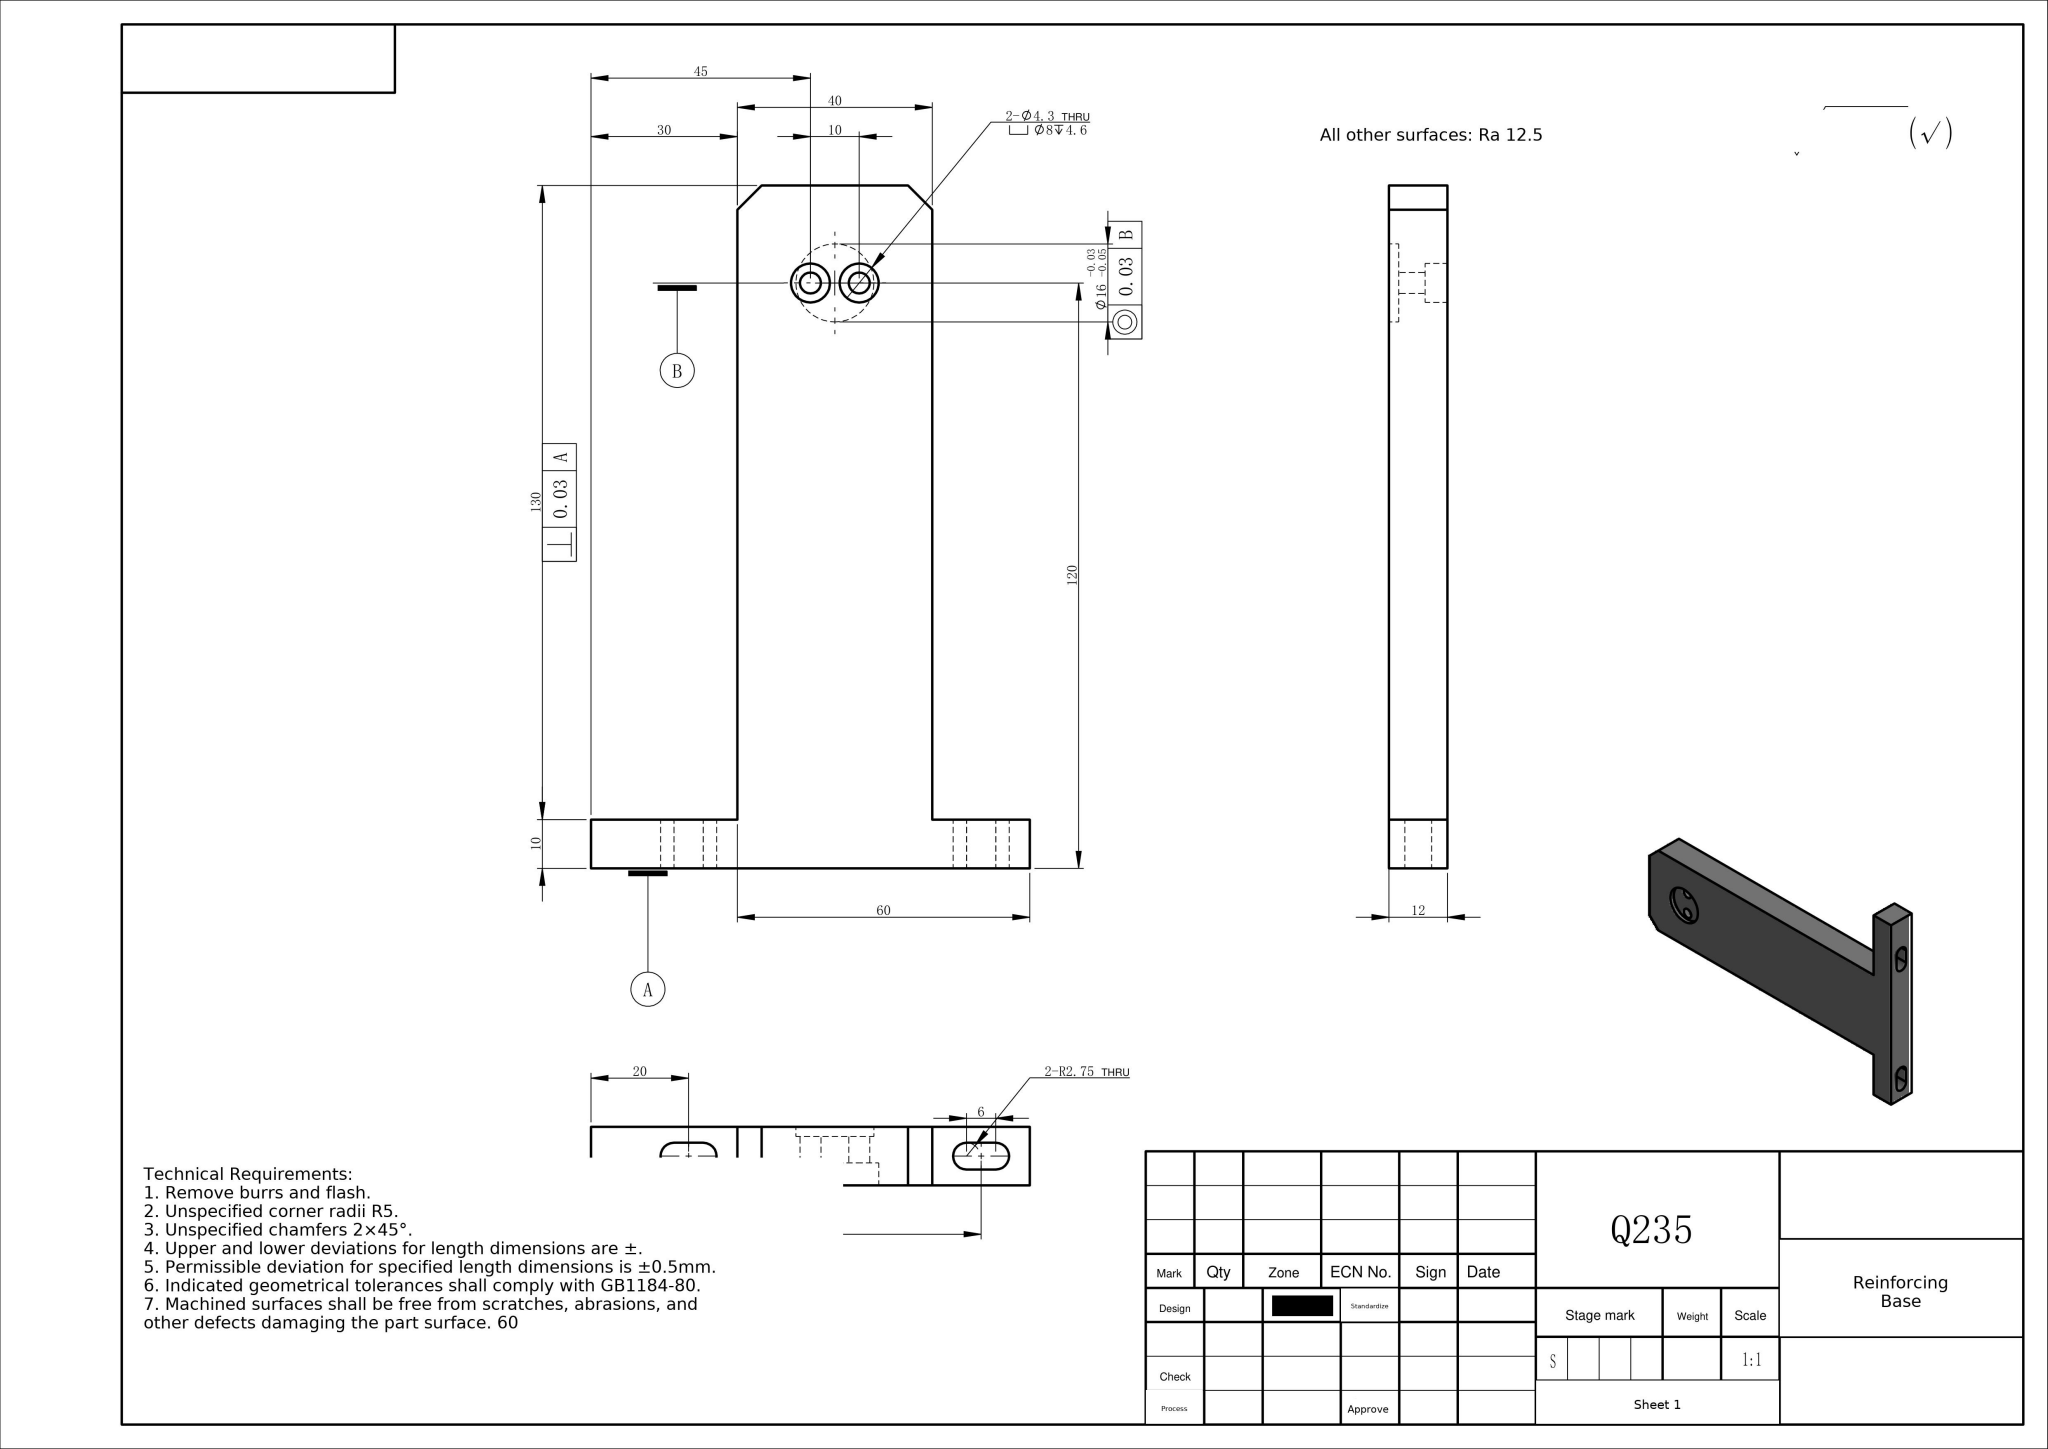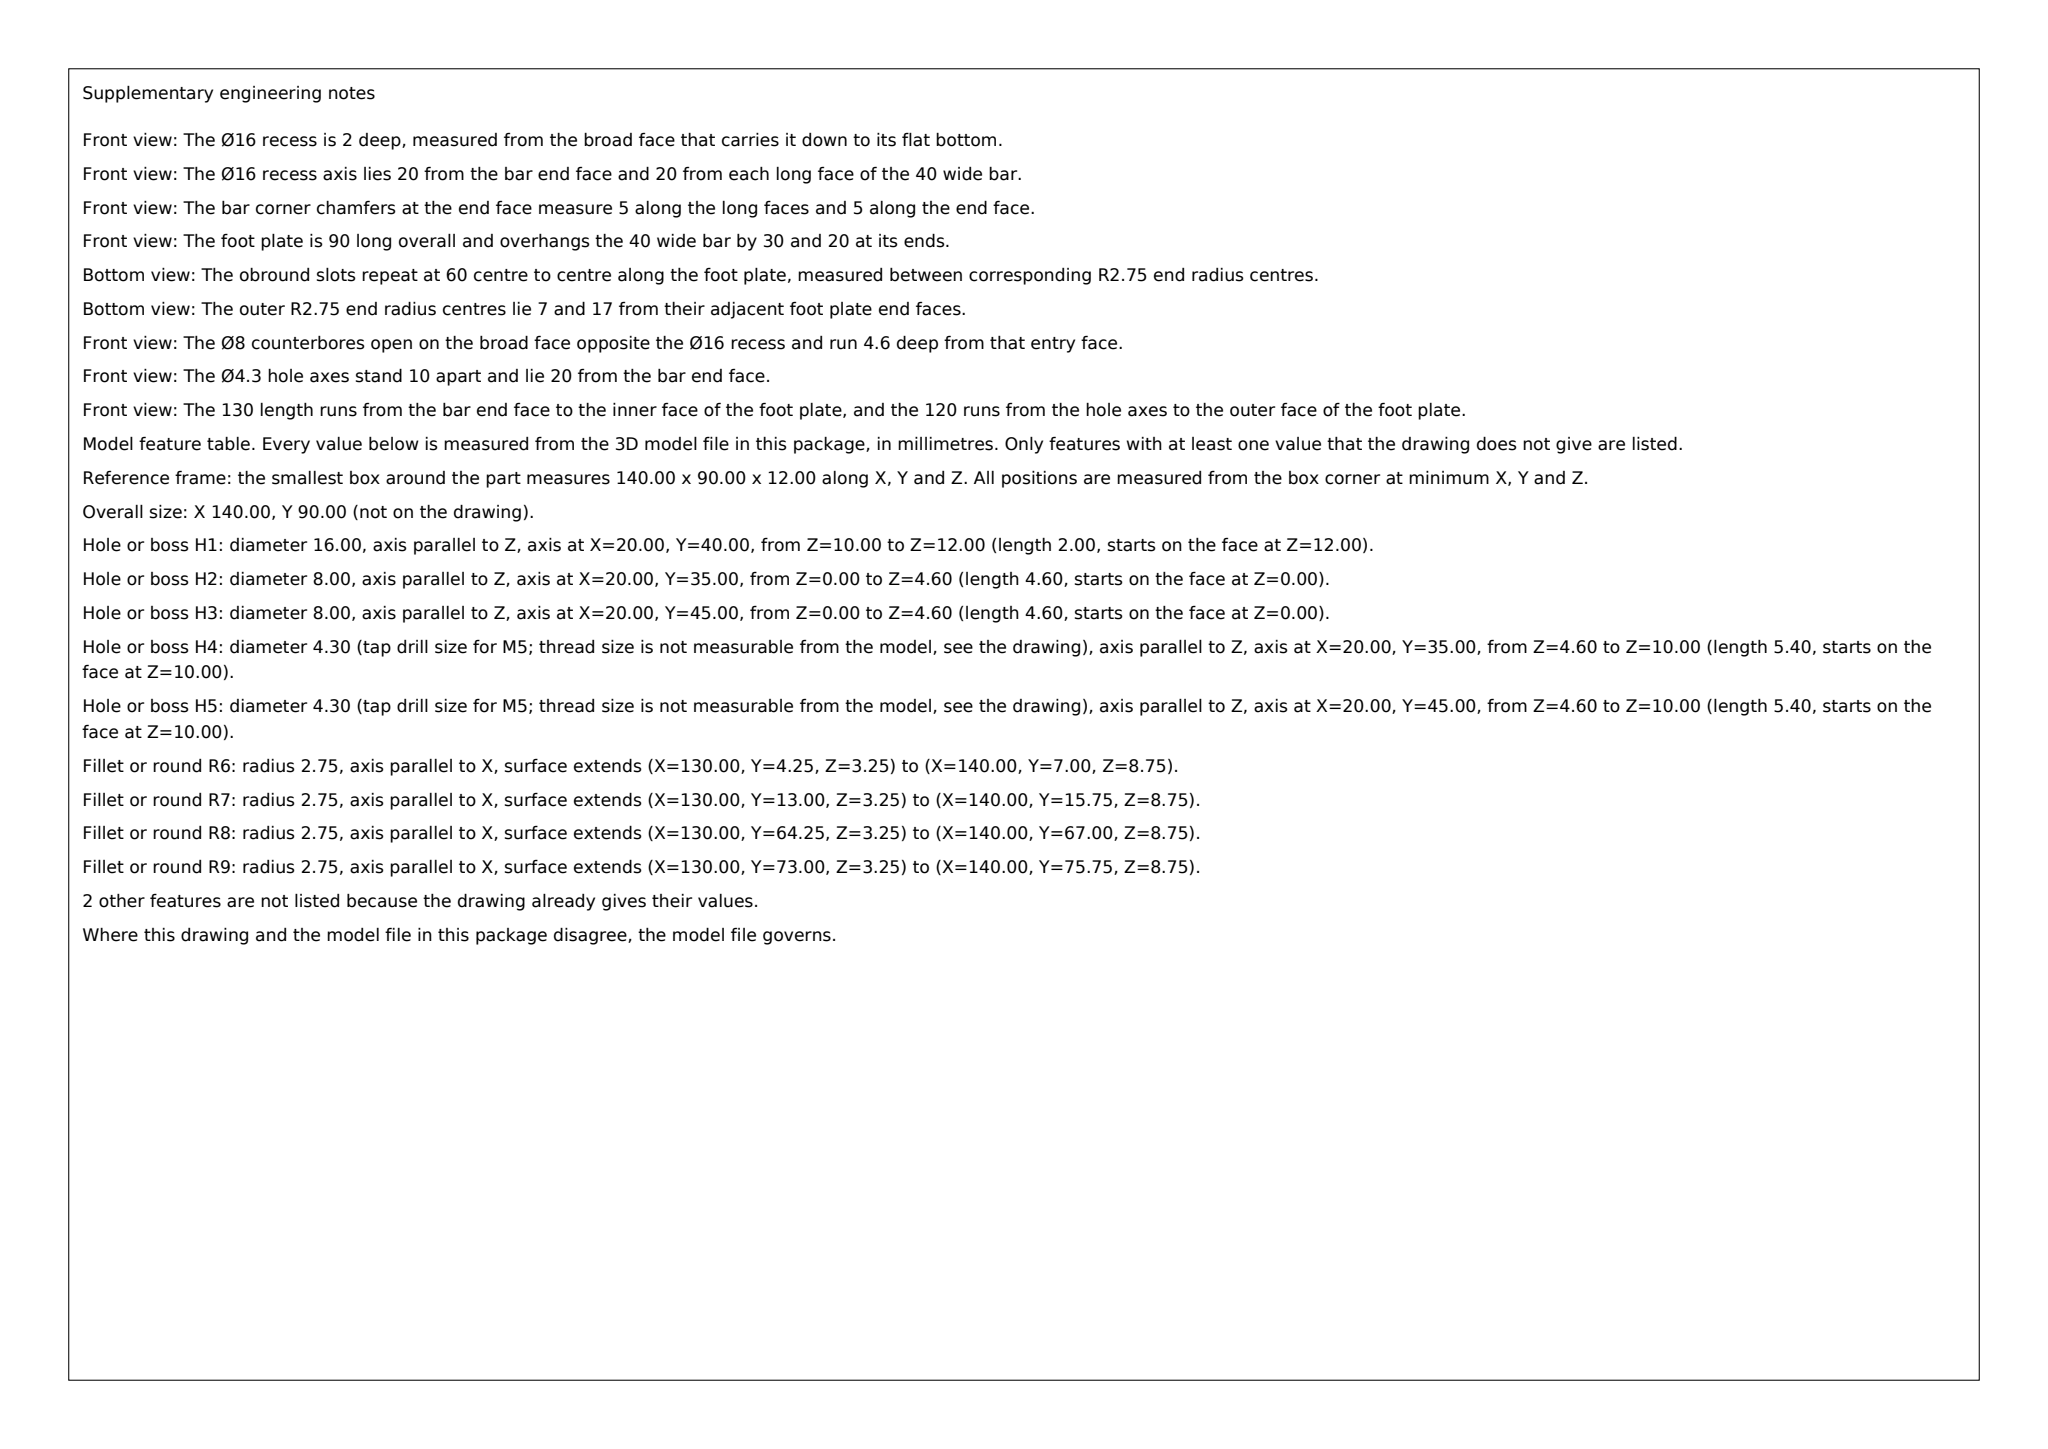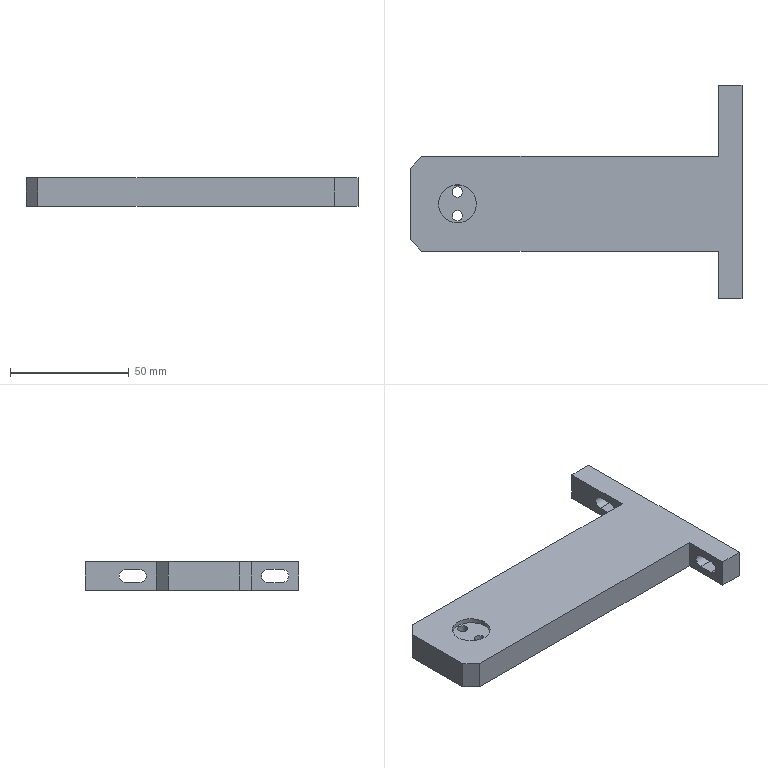Part | SolidWorks | mm | 1 solid | 35 faces | box 140 x 90 x 12 mm | volume 70743 mm3 | plane 19 | cylinder 16 | commonest cylinder face diameters 5.5 x6 4.3 x4 8 x4 16 x2
Drawing notes:
BTM VIEW: 2-R2.75 SLOTS 60 BETWEEN CTRS, 2ND CTR 10 FROM EDGE | from the solid: R2.75 (dia 5.5) x-axis holes at y=7,13 and y=67,73; plate y=0..90, so slot ctrs y=10 & y=70 -> 60 apart, 10 and 20 from edges